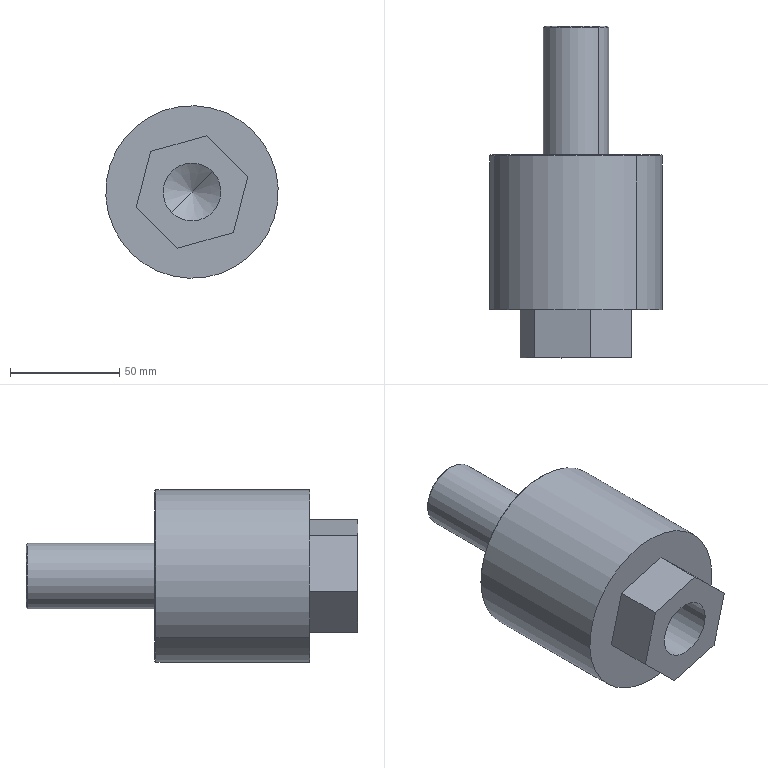Component | SolidWorks | FloatingJointJA140-30-150-1 | 1 solid | 22 faces | box 79 x 152 x 79 mm | volume 405367 mm3 | plane 10 | cylinder 6 | cone 6 | commonest cylinder face diameters 26.5 x2 79 x2 30 x2
STEP:
#1=CARTESIAN_POINT('',(-3.638,47.083,27.291));
#2=VERTEX_POINT('',#1);
#3=CARTESIAN_POINT('',(-4.368,47.083,26.546));
#4=VERTEX_POINT('',#3);
#5=CARTESIAN_POINT('',(-4.003,47.083,26.918));
#6=DIRECTION('',(-0.,-1.,0.));
#7=DIRECTION('',(-0.7002,0.,-0.7139));
#8=AXIS2_PLACEMENT_3D('',#5,#6,#7);
#9=CIRCLE('',#8,0.5217);
#10=EDGE_CURVE('',#2,#4,#9,.T.);
#11=ORIENTED_EDGE('',*,*,#10,.F.);
#12=CARTESIAN_POINT('',(-3.638,45.429,27.291));
#13=VERTEX_POINT('',#12);
#14=CARTESIAN_POINT('',(-3.638,45.429,27.291));
#15=DIRECTION('',(-0.,-1.,0.));
#16=VECTOR('',#15,39.37);
#17=LINE('',#14,#16);
#18=EDGE_CURVE('',#2,#13,#17,.T.);
#19=ORIENTED_EDGE('',*,*,#18,.T.);
#20=CARTESIAN_POINT('',(-4.368,45.429,26.546));
#21=VERTEX_POINT('',#20);
#22=CARTESIAN_POINT('',(-4.003,45.429,26.918));
#23=DIRECTION('',(-0.,-1.,0.));
#24=DIRECTION('',(-0.7002,0.,-0.7139));
#25=AXIS2_PLACEMENT_3D('',#22,#23,#24);
#26=CIRCLE('',#25,0.5217);
#27=EDGE_CURVE('',#13,#21,#26,.T.);
#28=ORIENTED_EDGE('',*,*,#27,.T.);
#29=CARTESIAN_POINT('',(-4.368,45.429,26.546));
#30=DIRECTION('',(-0.,-1.,0.));
#31=VECTOR('',#30,39.37);
#32=LINE('',#29,#31);
#33=EDGE_CURVE('',#4,#21,#32,.T.);
#34=ORIENTED_EDGE('',*,*,#33,.F.);
#35=EDGE_LOOP('',(#11,#19,#28,#34));
#36=FACE_OUTER_BOUND('',#35,.T.);
#37=CARTESIAN_POINT('',(-4.003,45.429,26.918));
#38=DIRECTION('',(-0.,-1.,0.));
#39=DIRECTION('',(-0.7002,0.,-0.7139));
#40=AXIS2_PLACEMENT_3D('',#37,#38,#39);
#41=CYLINDRICAL_SURFACE('',#40,0.5217);
#42=ADVANCED_FACE('',(#36),#41,.F.);
#43=CARTESIAN_POINT('',(-4.003,47.396,26.918));
#44=VERTEX_POINT('',#43);
#45=CARTESIAN_POINT('',(-4.368,47.083,26.546));
#46=DIRECTION('',(-0.6002,-0.515,-0.6119));
#47=VECTOR('',#46,39.37);
#48=LINE('',#45,#47);
#49=EDGE_CURVE('',#44,#4,#48,.T.);
#50=ORIENTED_EDGE('',*,*,#49,.F.);
#51=CARTESIAN_POINT('',(-3.638,47.083,27.291));
#52=DIRECTION('',(0.6002,-0.515,0.6119));
#53=VECTOR('',#52,39.37);
#54=LINE('',#51,#53);
#55=EDGE_CURVE('',#44,#2,#54,.T.);
#56=ORIENTED_EDGE('',*,*,#55,.T.);
#57=ORIENTED_EDGE('',*,*,#10,.T.);
#58=EDGE_LOOP('',(#50,#56,#57));
#59=FACE_OUTER_BOUND('',#58,.T.);
#60=CARTESIAN_POINT('',(-4.003,47.083,26.918));
#61=DIRECTION('',(-0.,-1.,0.));
#62=DIRECTION('',(-0.7002,0.,-0.7139));
#63=AXIS2_PLACEMENT_3D('',#60,#61,#62);
#64=CONICAL_SURFACE('',#63,0.5217,1.03);
#65=ADVANCED_FACE('',(#59),#64,.F.);
#66=CARTESIAN_POINT('',(-3.603,51.413,27.326));
#67=VERTEX_POINT('',#66);
#68=CARTESIAN_POINT('',(-4.403,51.413,26.511));
#69=VERTEX_POINT('',#68);
#70=CARTESIAN_POINT('',(-4.003,51.413,26.918));
#71=DIRECTION('',(0.,1.,-0.));
#72=DIRECTION('',(0.7002,0.,0.7139));
#73=AXIS2_PLACEMENT_3D('',#70,#71,#72);
#74=CIRCLE('',#73,0.5709);
#75=EDGE_CURVE('',#67,#69,#74,.T.);
#76=ORIENTED_EDGE('',*,*,#75,.F.);
#77=CARTESIAN_POINT('',(-3.59,51.394,27.34));
#78=VERTEX_POINT('',#77);
#79=CARTESIAN_POINT('',(-3.59,51.394,27.34));
#80=DIRECTION('',(0.4951,-0.7071,0.5048));
#81=VECTOR('',#80,39.37);
#82=LINE('',#79,#81);
#83=EDGE_CURVE('',#67,#78,#82,.T.);
#84=ORIENTED_EDGE('',*,*,#83,.T.);
#85=CARTESIAN_POINT('',(-4.417,51.394,26.497));
#86=VERTEX_POINT('',#85);
#87=CARTESIAN_POINT('',(-4.003,51.394,26.918));
#88=DIRECTION('',(-0.,-1.,0.));
#89=DIRECTION('',(0.7002,0.,0.7139));
#90=AXIS2_PLACEMENT_3D('',#87,#88,#89);
#91=CIRCLE('',#90,0.5906);
#92=EDGE_CURVE('',#86,#78,#91,.T.);
#93=ORIENTED_EDGE('',*,*,#92,.F.);
#94=CARTESIAN_POINT('',(-4.417,51.394,26.497));
#95=DIRECTION('',(-0.4951,-0.7071,-0.5048));
#96=VECTOR('',#95,39.37);
#97=LINE('',#94,#96);
#98=EDGE_CURVE('',#69,#86,#97,.T.);
#99=ORIENTED_EDGE('',*,*,#98,.F.);
#100=EDGE_LOOP('',(#76,#84,#93,#99));
#101=FACE_OUTER_BOUND('',#100,.T.);
#102=CARTESIAN_POINT('',(-4.003,51.394,26.918));
#103=DIRECTION('',(-0.,-1.,0.));
#104=DIRECTION('',(-0.7002,0.,-0.7139));
#105=AXIS2_PLACEMENT_3D('',#102,#103,#104);
#106=CONICAL_SURFACE('',#105,0.5906,0.7854);
#107=ADVANCED_FACE('',(#101),#106,.T.);
#108=CARTESIAN_POINT('',(-2.928,49.09,28.014));
#109=VERTEX_POINT('',#108);
#110=CARTESIAN_POINT('',(-5.078,49.09,25.822));
#111=VERTEX_POINT('',#110);
#112=CARTESIAN_POINT('',(-4.003,49.09,26.918));
#113=DIRECTION('',(0.,1.,-0.));
#114=DIRECTION('',(0.7002,0.,0.7139));
#115=AXIS2_PLACEMENT_3D('',#112,#113,#114);
#116=CIRCLE('',#115,1.535);
#117=EDGE_CURVE('',#109,#111,#116,.T.);
#118=ORIENTED_EDGE('',*,*,#117,.F.);
#119=CARTESIAN_POINT('',(-2.914,49.071,28.028));
#120=VERTEX_POINT('',#119);
#121=CARTESIAN_POINT('',(-2.914,49.071,28.028));
#122=DIRECTION('',(0.4951,-0.7071,0.5048));
#123=VECTOR('',#122,39.37);
#124=LINE('',#121,#123);
#125=EDGE_CURVE('',#109,#120,#124,.T.);
#126=ORIENTED_EDGE('',*,*,#125,.T.);
#127=CARTESIAN_POINT('',(-5.092,49.071,25.808));
#128=VERTEX_POINT('',#127);
#129=CARTESIAN_POINT('',(-4.003,49.071,26.918));
#130=DIRECTION('',(-0.,-1.,0.));
#131=DIRECTION('',(0.7002,0.,0.7139));
#132=AXIS2_PLACEMENT_3D('',#129,#130,#131);
#133=CIRCLE('',#132,1.555);
#134=EDGE_CURVE('',#128,#120,#133,.T.);
#135=ORIENTED_EDGE('',*,*,#134,.F.);
#136=CARTESIAN_POINT('',(-5.092,49.071,25.808));
#137=DIRECTION('',(-0.4951,-0.7071,-0.5048));
#138=VECTOR('',#137,39.37);
#139=LINE('',#136,#138);
#140=EDGE_CURVE('',#111,#128,#139,.T.);
#141=ORIENTED_EDGE('',*,*,#140,.F.);
#142=EDGE_LOOP('',(#118,#126,#135,#141));
#143=FACE_OUTER_BOUND('',#142,.T.);
#144=CARTESIAN_POINT('',(-4.003,49.071,26.918));
#145=DIRECTION('',(-0.,-1.,0.));
#146=DIRECTION('',(-0.7002,0.,-0.7139));
#147=AXIS2_PLACEMENT_3D('',#144,#145,#146);
#148=CONICAL_SURFACE('',#147,1.555,0.7854);
#149=ADVANCED_FACE('',(#143),#148,.T.);
#150=ORIENTED_EDGE('',*,*,#134,.T.);
#151=CARTESIAN_POINT('',(-2.914,46.295,28.028));
#152=VERTEX_POINT('',#151);
#153=CARTESIAN_POINT('',(-2.914,45.429,28.028));
#154=DIRECTION('',(-0.,-1.,0.));
#155=VECTOR('',#154,39.37);
#156=LINE('',#153,#155);
#157=EDGE_CURVE('',#120,#152,#156,.T.);
#158=ORIENTED_EDGE('',*,*,#157,.T.);
#159=CARTESIAN_POINT('',(-5.092,46.295,25.808));
#160=VERTEX_POINT('',#159);
#161=CARTESIAN_POINT('',(-4.003,46.295,26.918));
#162=DIRECTION('',(-0.,-1.,0.));
#163=DIRECTION('',(-0.7002,0.,-0.7139));
#164=AXIS2_PLACEMENT_3D('',#161,#162,#163);
#165=CIRCLE('',#164,1.555);
#166=EDGE_CURVE('',#160,#152,#165,.T.);
#167=ORIENTED_EDGE('',*,*,#166,.F.);
#168=CARTESIAN_POINT('',(-5.092,45.429,25.808));
#169=DIRECTION('',(-0.,-1.,0.));
#170=VECTOR('',#169,39.37);
#171=LINE('',#168,#170);
#172=EDGE_CURVE('',#128,#160,#171,.T.);
#173=ORIENTED_EDGE('',*,*,#172,.F.);
#174=EDGE_LOOP('',(#150,#158,#167,#173));
#175=FACE_OUTER_BOUND('',#174,.T.);
#176=CARTESIAN_POINT('',(-4.003,45.429,26.918));
#177=DIRECTION('',(-0.,-1.,0.));
#178=DIRECTION('',(-0.7002,0.,-0.7139));
#179=AXIS2_PLACEMENT_3D('',#176,#177,#178);
#180=CYLINDRICAL_SURFACE('',#179,1.555);
#181=ADVANCED_FACE('',(#175),#180,.T.);
#182=ORIENTED_EDGE('',*,*,#92,.T.);
#183=CARTESIAN_POINT('',(-3.59,49.09,27.34));
#184=VERTEX_POINT('',#183);
#185=CARTESIAN_POINT('',(-3.59,45.429,27.34));
#186=DIRECTION('',(-0.,-1.,0.));
#187=VECTOR('',#186,39.37);
#188=LINE('',#185,#187);
#189=EDGE_CURVE('',#78,#184,#188,.T.);
#190=ORIENTED_EDGE('',*,*,#189,.T.);
#191=CARTESIAN_POINT('',(-4.417,49.09,26.497));
#192=VERTEX_POINT('',#191);
#193=CARTESIAN_POINT('',(-4.003,49.09,26.918));
#194=DIRECTION('',(-0.,-1.,0.));
#195=DIRECTION('',(-0.7002,0.,-0.7139));
#196=AXIS2_PLACEMENT_3D('',#193,#194,#195);
#197=CIRCLE('',#196,0.5906);
#198=EDGE_CURVE('',#192,#184,#197,.T.);
#199=ORIENTED_EDGE('',*,*,#198,.F.);
#200=CARTESIAN_POINT('',(-4.417,45.429,26.497));
#201=DIRECTION('',(-0.,-1.,0.));
#202=VECTOR('',#201,39.37);
#203=LINE('',#200,#202);
#204=EDGE_CURVE('',#86,#192,#203,.T.);
#205=ORIENTED_EDGE('',*,*,#204,.F.);
#206=EDGE_LOOP('',(#182,#190,#199,#205));
#207=FACE_OUTER_BOUND('',#206,.T.);
#208=CARTESIAN_POINT('',(-4.003,45.429,26.918));
#209=DIRECTION('',(-0.,-1.,0.));
#210=DIRECTION('',(-0.7002,0.,-0.7139));
#211=AXIS2_PLACEMENT_3D('',#208,#209,#210);
#212=CYLINDRICAL_SURFACE('',#211,0.5906);
#213=ADVANCED_FACE('',(#207),#212,.T.);
#214=CARTESIAN_POINT('',(-4.003,51.413,26.918));
#215=DIRECTION('',(0.,1.,-0.));
#216=DIRECTION('',(0.7002,0.,0.7139));
#217=AXIS2_PLACEMENT_3D('',#214,#215,#216);
#218=CIRCLE('',#217,0.5709);
#219=EDGE_CURVE('',#69,#67,#218,.T.);
#220=ORIENTED_EDGE('',*,*,#219,.T.);
#221=ORIENTED_EDGE('',*,*,#75,.T.);
#222=EDGE_LOOP('',(#220,#221));
#223=FACE_OUTER_BOUND('',#222,.T.);
#224=CARTESIAN_POINT('',(-4.003,51.413,26.918));
#225=DIRECTION('',(0.,1.,-0.));
#226=DIRECTION('',(0.7002,-0.,0.7139));
#227=AXIS2_PLACEMENT_3D('',#224,#225,#226);
#228=PLANE('',#227);
#229=ADVANCED_FACE('',(#223),#228,.T.);
#230=ORIENTED_EDGE('',*,*,#189,.F.);
#231=CARTESIAN_POINT('',(-4.003,51.394,26.918));
#232=DIRECTION('',(-0.,-1.,0.));
#233=DIRECTION('',(0.7002,0.,0.7139));
#234=AXIS2_PLACEMENT_3D('',#231,#232,#233);
#235=CIRCLE('',#234,0.5906);
#236=EDGE_CURVE('',#78,#86,#235,.T.);
#237=ORIENTED_EDGE('',*,*,#236,.T.);
#238=ORIENTED_EDGE('',*,*,#204,.T.);
#239=CARTESIAN_POINT('',(-4.003,49.09,26.918));
#240=DIRECTION('',(-0.,-1.,0.));
#241=DIRECTION('',(-0.7002,0.,-0.7139));
#242=AXIS2_PLACEMENT_3D('',#239,#240,#241);
#243=CIRCLE('',#242,0.5906);
#244=EDGE_CURVE('',#184,#192,#243,.T.);
#245=ORIENTED_EDGE('',*,*,#244,.F.);
#246=EDGE_LOOP('',(#230,#237,#238,#245));
#247=FACE_OUTER_BOUND('',#246,.T.);
#248=CARTESIAN_POINT('',(-4.003,45.429,26.918));
#249=DIRECTION('',(-0.,-1.,0.));
#250=DIRECTION('',(-0.7002,0.,-0.7139));
#251=AXIS2_PLACEMENT_3D('',#248,#249,#250);
#252=CYLINDRICAL_SURFACE('',#251,0.5906);
#253=ADVANCED_FACE('',(#247),#252,.T.);
#254=CARTESIAN_POINT('',(-4.003,49.09,26.918));
#255=DIRECTION('',(0.,1.,-0.));
#256=DIRECTION('',(0.7002,0.,0.7139));
#257=AXIS2_PLACEMENT_3D('',#254,#255,#256);
#258=CIRCLE('',#257,1.535);
#259=EDGE_CURVE('',#111,#109,#258,.T.);
#260=ORIENTED_EDGE('',*,*,#259,.T.);
#261=ORIENTED_EDGE('',*,*,#117,.T.);
#262=EDGE_LOOP('',(#260,#261));
#263=FACE_OUTER_BOUND('',#262,.T.);
#264=ORIENTED_EDGE('',*,*,#198,.T.);
#265=ORIENTED_EDGE('',*,*,#244,.T.);
#266=EDGE_LOOP('',(#264,#265));
#267=FACE_BOUND('',#266,.T.);
#268=CARTESIAN_POINT('',(-5.092,49.09,25.808));
#269=DIRECTION('',(0.,1.,-0.));
#270=DIRECTION('',(0.7002,-0.,0.7139));
#271=AXIS2_PLACEMENT_3D('',#268,#269,#270);
#272=PLANE('',#271);
#273=ADVANCED_FACE('',(#263,#267),#272,.T.);
#274=ORIENTED_EDGE('',*,*,#157,.F.);
#275=CARTESIAN_POINT('',(-4.003,49.071,26.918));
#276=DIRECTION('',(-0.,-1.,0.));
#277=DIRECTION('',(0.7002,0.,0.7139));
#278=AXIS2_PLACEMENT_3D('',#275,#276,#277);
#279=CIRCLE('',#278,1.555);
#280=EDGE_CURVE('',#120,#128,#279,.T.);
#281=ORIENTED_EDGE('',*,*,#280,.T.);
#282=ORIENTED_EDGE('',*,*,#172,.T.);
#283=CARTESIAN_POINT('',(-4.003,46.295,26.918));
#284=DIRECTION('',(-0.,-1.,0.));
#285=DIRECTION('',(-0.7002,0.,-0.7139));
#286=AXIS2_PLACEMENT_3D('',#283,#284,#285);
#287=CIRCLE('',#286,1.555);
#288=EDGE_CURVE('',#152,#160,#287,.T.);
#289=ORIENTED_EDGE('',*,*,#288,.F.);
#290=EDGE_LOOP('',(#274,#281,#282,#289));
#291=FACE_OUTER_BOUND('',#290,.T.);
#292=CARTESIAN_POINT('',(-4.003,45.429,26.918));
#293=DIRECTION('',(-0.,-1.,0.));
#294=DIRECTION('',(-0.7002,0.,-0.7139));
#295=AXIS2_PLACEMENT_3D('',#292,#293,#294);
#296=CYLINDRICAL_SURFACE('',#295,1.555);
#297=ADVANCED_FACE('',(#291),#296,.T.);
#298=ORIENTED_EDGE('',*,*,#166,.T.);
#299=ORIENTED_EDGE('',*,*,#288,.T.);
#300=EDGE_LOOP('',(#298,#299));
#301=FACE_OUTER_BOUND('',#300,.T.);
#302=CARTESIAN_POINT('',(-4.264,46.295,25.906));
#303=VERTEX_POINT('',#302);
#304=CARTESIAN_POINT('',(-3.257,46.295,26.186));
#305=VERTEX_POINT('',#304);
#306=CARTESIAN_POINT('',(-4.264,46.295,25.906));
#307=DIRECTION('',(0.9634,0.,0.2682));
#308=VECTOR('',#307,39.37);
#309=LINE('',#306,#308);
#310=EDGE_CURVE('',#303,#305,#309,.T.);
#311=ORIENTED_EDGE('',*,*,#310,.F.);
#312=CARTESIAN_POINT('',(-5.01,46.295,26.638));
#313=VERTEX_POINT('',#312);
#314=CARTESIAN_POINT('',(-5.01,46.295,26.638));
#315=DIRECTION('',(0.7139,0.,-0.7002));
#316=VECTOR('',#315,39.37);
#317=LINE('',#314,#316);
#318=EDGE_CURVE('',#313,#303,#317,.T.);
#319=ORIENTED_EDGE('',*,*,#318,.F.);
#320=CARTESIAN_POINT('',(-4.75,46.295,27.65));
#321=VERTEX_POINT('',#320);
#322=CARTESIAN_POINT('',(-4.75,46.295,27.65));
#323=DIRECTION('',(-0.2495,0.,-0.9684));
#324=VECTOR('',#323,39.37);
#325=LINE('',#322,#324);
#326=EDGE_CURVE('',#321,#313,#325,.T.);
#327=ORIENTED_EDGE('',*,*,#326,.F.);
#328=CARTESIAN_POINT('',(-3.742,46.295,27.931));
#329=VERTEX_POINT('',#328);
#330=CARTESIAN_POINT('',(-3.742,46.295,27.931));
#331=DIRECTION('',(-0.9634,-0.,-0.2682));
#332=VECTOR('',#331,39.37);
#333=LINE('',#330,#332);
#334=EDGE_CURVE('',#329,#321,#333,.T.);
#335=ORIENTED_EDGE('',*,*,#334,.F.);
#336=CARTESIAN_POINT('',(-2.996,46.295,27.199));
#337=VERTEX_POINT('',#336);
#338=CARTESIAN_POINT('',(-2.996,46.295,27.199));
#339=DIRECTION('',(-0.7139,-0.,0.7002));
#340=VECTOR('',#339,39.37);
#341=LINE('',#338,#340);
#342=EDGE_CURVE('',#337,#329,#341,.T.);
#343=ORIENTED_EDGE('',*,*,#342,.F.);
#344=CARTESIAN_POINT('',(-3.257,46.295,26.186));
#345=DIRECTION('',(0.2495,-0.,0.9684));
#346=VECTOR('',#345,39.37);
#347=LINE('',#344,#346);
#348=EDGE_CURVE('',#305,#337,#347,.T.);
#349=ORIENTED_EDGE('',*,*,#348,.F.);
#350=EDGE_LOOP('',(#311,#319,#327,#335,#343,#349));
#351=FACE_BOUND('',#350,.T.);
#352=CARTESIAN_POINT('',(-5.092,46.295,25.808));
#353=DIRECTION('',(-0.,-1.,0.));
#354=DIRECTION('',(-0.7002,0.,-0.7139));
#355=AXIS2_PLACEMENT_3D('',#352,#353,#354);
#356=PLANE('',#355);
#357=ADVANCED_FACE('',(#301,#351),#356,.T.);
#358=CARTESIAN_POINT('',(-3.257,45.429,26.186));
#359=VERTEX_POINT('',#358);
#360=CARTESIAN_POINT('',(-4.264,45.429,25.906));
#361=VERTEX_POINT('',#360);
#362=CARTESIAN_POINT('',(-4.91,45.429,25.726));
#363=DIRECTION('',(-0.9634,-0.,-0.2682));
#364=VECTOR('',#363,39.37);
#365=LINE('',#362,#364);
#366=EDGE_CURVE('',#359,#361,#365,.T.);
#367=ORIENTED_EDGE('',*,*,#366,.T.);
#368=CARTESIAN_POINT('',(-4.264,44.72,25.906));
#369=DIRECTION('',(0.,1.,-0.));
#370=VECTOR('',#369,39.37);
#371=LINE('',#368,#370);
#372=EDGE_CURVE('',#361,#303,#371,.T.);
#373=ORIENTED_EDGE('',*,*,#372,.T.);
#374=ORIENTED_EDGE('',*,*,#310,.T.);
#375=CARTESIAN_POINT('',(-3.257,44.72,26.186));
#376=DIRECTION('',(0.,1.,-0.));
#377=VECTOR('',#376,39.37);
#378=LINE('',#375,#377);
#379=EDGE_CURVE('',#359,#305,#378,.T.);
#380=ORIENTED_EDGE('',*,*,#379,.F.);
#381=EDGE_LOOP('',(#367,#373,#374,#380));
#382=FACE_OUTER_BOUND('',#381,.T.);
#383=CARTESIAN_POINT('',(-4.264,44.72,25.906));
#384=DIRECTION('',(-0.2682,-0.,0.9634));
#385=DIRECTION('',(-0.9634,-0.,-0.2682));
#386=AXIS2_PLACEMENT_3D('',#383,#384,#385);
#387=PLANE('',#386);
#388=ADVANCED_FACE('',(#382),#387,.F.);
#389=CARTESIAN_POINT('',(-2.996,45.429,27.199));
#390=VERTEX_POINT('',#389);
#391=CARTESIAN_POINT('',(-3.424,45.429,25.537));
#392=DIRECTION('',(-0.2495,0.,-0.9684));
#393=VECTOR('',#392,39.37);
#394=LINE('',#391,#393);
#395=EDGE_CURVE('',#390,#359,#394,.T.);
#396=ORIENTED_EDGE('',*,*,#395,.T.);
#397=ORIENTED_EDGE('',*,*,#379,.T.);
#398=ORIENTED_EDGE('',*,*,#348,.T.);
#399=CARTESIAN_POINT('',(-2.996,44.72,27.199));
#400=DIRECTION('',(0.,1.,-0.));
#401=VECTOR('',#400,39.37);
#402=LINE('',#399,#401);
#403=EDGE_CURVE('',#390,#337,#402,.T.);
#404=ORIENTED_EDGE('',*,*,#403,.F.);
#405=EDGE_LOOP('',(#396,#397,#398,#404));
#406=FACE_OUTER_BOUND('',#405,.T.);
#407=CARTESIAN_POINT('',(-3.257,44.72,26.186));
#408=DIRECTION('',(-0.9684,-0.,0.2495));
#409=DIRECTION('',(-0.2495,0.,-0.9684));
#410=AXIS2_PLACEMENT_3D('',#407,#408,#409);
#411=PLANE('',#410);
#412=ADVANCED_FACE('',(#406),#411,.F.);
#413=CARTESIAN_POINT('',(-3.742,45.429,27.931));
#414=VERTEX_POINT('',#413);
#415=CARTESIAN_POINT('',(-3.369,45.429,27.565));
#416=DIRECTION('',(0.7139,0.,-0.7002));
#417=VECTOR('',#416,39.37);
#418=LINE('',#415,#417);
#419=EDGE_CURVE('',#414,#390,#418,.T.);
#420=ORIENTED_EDGE('',*,*,#419,.T.);
#421=ORIENTED_EDGE('',*,*,#403,.T.);
#422=ORIENTED_EDGE('',*,*,#342,.T.);
#423=CARTESIAN_POINT('',(-3.742,44.72,27.931));
#424=DIRECTION('',(0.,1.,-0.));
#425=VECTOR('',#424,39.37);
#426=LINE('',#423,#425);
#427=EDGE_CURVE('',#414,#329,#426,.T.);
#428=ORIENTED_EDGE('',*,*,#427,.F.);
#429=EDGE_LOOP('',(#420,#421,#422,#428));
#430=FACE_OUTER_BOUND('',#429,.T.);
#431=CARTESIAN_POINT('',(-2.996,44.72,27.199));
#432=DIRECTION('',(-0.7002,-0.,-0.7139));
#433=DIRECTION('',(0.,1.,-0.));
#434=AXIS2_PLACEMENT_3D('',#431,#432,#433);
#435=PLANE('',#434);
#436=ADVANCED_FACE('',(#430),#435,.F.);
#437=CARTESIAN_POINT('',(-4.75,45.429,27.65));
#438=VERTEX_POINT('',#437);
#439=CARTESIAN_POINT('',(-5.396,45.429,27.471));
#440=DIRECTION('',(0.9634,0.,0.2682));
#441=VECTOR('',#440,39.37);
#442=LINE('',#439,#441);
#443=EDGE_CURVE('',#438,#414,#442,.T.);
#444=ORIENTED_EDGE('',*,*,#443,.T.);
#445=ORIENTED_EDGE('',*,*,#427,.T.);
#446=ORIENTED_EDGE('',*,*,#334,.T.);
#447=CARTESIAN_POINT('',(-4.75,44.72,27.65));
#448=DIRECTION('',(0.,1.,-0.));
#449=VECTOR('',#448,39.37);
#450=LINE('',#447,#449);
#451=EDGE_CURVE('',#438,#321,#450,.T.);
#452=ORIENTED_EDGE('',*,*,#451,.F.);
#453=EDGE_LOOP('',(#444,#445,#446,#452));
#454=FACE_OUTER_BOUND('',#453,.T.);
#455=CARTESIAN_POINT('',(-3.742,44.72,27.931));
#456=DIRECTION('',(0.2682,0.,-0.9634));
#457=DIRECTION('',(0.9634,0.,0.2682));
#458=AXIS2_PLACEMENT_3D('',#455,#456,#457);
#459=PLANE('',#458);
#460=ADVANCED_FACE('',(#454),#459,.F.);
#461=CARTESIAN_POINT('',(-5.01,45.429,26.638));
#462=VERTEX_POINT('',#461);
#463=CARTESIAN_POINT('',(-5.178,45.429,25.988));
#464=DIRECTION('',(0.2495,-0.,0.9684));
#465=VECTOR('',#464,39.37);
#466=LINE('',#463,#465);
#467=EDGE_CURVE('',#462,#438,#466,.T.);
#468=ORIENTED_EDGE('',*,*,#467,.T.);
#469=ORIENTED_EDGE('',*,*,#451,.T.);
#470=ORIENTED_EDGE('',*,*,#326,.T.);
#471=CARTESIAN_POINT('',(-5.01,44.72,26.638));
#472=DIRECTION('',(0.,1.,-0.));
#473=VECTOR('',#472,39.37);
#474=LINE('',#471,#473);
#475=EDGE_CURVE('',#462,#313,#474,.T.);
#476=ORIENTED_EDGE('',*,*,#475,.F.);
#477=EDGE_LOOP('',(#468,#469,#470,#476));
#478=FACE_OUTER_BOUND('',#477,.T.);
#479=CARTESIAN_POINT('',(-4.75,44.72,27.65));
#480=DIRECTION('',(0.9684,0.,-0.2495));
#481=DIRECTION('',(0.2495,-0.,0.9684));
#482=AXIS2_PLACEMENT_3D('',#479,#480,#481);
#483=PLANE('',#482);
#484=ADVANCED_FACE('',(#478),#483,.F.);
#485=CARTESIAN_POINT('',(-4.637,45.429,26.272));
#486=DIRECTION('',(-0.7139,-0.,0.7002));
#487=VECTOR('',#486,39.37);
#488=LINE('',#485,#487);
#489=EDGE_CURVE('',#361,#462,#488,.T.);
#490=ORIENTED_EDGE('',*,*,#489,.T.);
#491=ORIENTED_EDGE('',*,*,#475,.T.);
#492=ORIENTED_EDGE('',*,*,#318,.T.);
#493=ORIENTED_EDGE('',*,*,#372,.F.);
#494=EDGE_LOOP('',(#490,#491,#492,#493));
#495=FACE_OUTER_BOUND('',#494,.T.);
#496=CARTESIAN_POINT('',(-5.01,44.72,26.638));
#497=DIRECTION('',(0.7002,0.,0.7139));
#498=DIRECTION('',(-0.,-1.,0.));
#499=AXIS2_PLACEMENT_3D('',#496,#497,#498);
#500=PLANE('',#499);
#501=ADVANCED_FACE('',(#495),#500,.F.);
#502=CARTESIAN_POINT('',(-4.003,45.429,26.918));
#503=DIRECTION('',(-0.,-1.,0.));
#504=DIRECTION('',(-0.7002,0.,-0.7139));
#505=AXIS2_PLACEMENT_3D('',#502,#503,#504);
#506=CIRCLE('',#505,0.5217);
#507=EDGE_CURVE('',#21,#13,#506,.T.);
#508=ORIENTED_EDGE('',*,*,#507,.F.);
#509=ORIENTED_EDGE('',*,*,#27,.F.);
#510=EDGE_LOOP('',(#508,#509));
#511=FACE_BOUND('',#510,.T.);
#512=ORIENTED_EDGE('',*,*,#366,.F.);
#513=ORIENTED_EDGE('',*,*,#395,.F.);
#514=ORIENTED_EDGE('',*,*,#419,.F.);
#515=ORIENTED_EDGE('',*,*,#443,.F.);
#516=ORIENTED_EDGE('',*,*,#467,.F.);
#517=ORIENTED_EDGE('',*,*,#489,.F.);
#518=EDGE_LOOP('',(#512,#513,#514,#515,#516,#517));
#519=FACE_OUTER_BOUND('',#518,.T.);
#520=CARTESIAN_POINT('',(-4.968,45.429,25.934));
#521=DIRECTION('',(-0.,-1.,0.));
#522=DIRECTION('',(-0.7002,0.,-0.7139));
#523=AXIS2_PLACEMENT_3D('',#520,#521,#522);
#524=PLANE('',#523);
#525=ADVANCED_FACE('',(#511,#519),#524,.T.);
#526=ORIENTED_EDGE('',*,*,#125,.F.);
#527=ORIENTED_EDGE('',*,*,#259,.F.);
#528=ORIENTED_EDGE('',*,*,#140,.T.);
#529=ORIENTED_EDGE('',*,*,#280,.F.);
#530=EDGE_LOOP('',(#526,#527,#528,#529));
#531=FACE_OUTER_BOUND('',#530,.T.);
#532=CARTESIAN_POINT('',(-4.003,49.071,26.918));
#533=DIRECTION('',(-0.,-1.,0.));
#534=DIRECTION('',(-0.7002,0.,-0.7139));
#535=AXIS2_PLACEMENT_3D('',#532,#533,#534);
#536=CONICAL_SURFACE('',#535,1.555,0.7854);
#537=ADVANCED_FACE('',(#531),#536,.T.);
#538=ORIENTED_EDGE('',*,*,#83,.F.);
#539=ORIENTED_EDGE('',*,*,#219,.F.);
#540=ORIENTED_EDGE('',*,*,#98,.T.);
#541=ORIENTED_EDGE('',*,*,#236,.F.);
#542=EDGE_LOOP('',(#538,#539,#540,#541));
#543=FACE_OUTER_BOUND('',#542,.T.);
#544=CARTESIAN_POINT('',(-4.003,51.394,26.918));
#545=DIRECTION('',(-0.,-1.,0.));
#546=DIRECTION('',(-0.7002,0.,-0.7139));
#547=AXIS2_PLACEMENT_3D('',#544,#545,#546);
#548=CONICAL_SURFACE('',#547,0.5906,0.7854);
#549=ADVANCED_FACE('',(#543),#548,.T.);
#550=ORIENTED_EDGE('',*,*,#55,.F.);
#551=ORIENTED_EDGE('',*,*,#49,.T.);
#552=CARTESIAN_POINT('',(-4.003,47.083,26.918));
#553=DIRECTION('',(-0.,-1.,0.));
#554=DIRECTION('',(-0.7002,0.,-0.7139));
#555=AXIS2_PLACEMENT_3D('',#552,#553,#554);
#556=CIRCLE('',#555,0.5217);
#557=EDGE_CURVE('',#4,#2,#556,.T.);
#558=ORIENTED_EDGE('',*,*,#557,.T.);
#559=EDGE_LOOP('',(#550,#551,#558));
#560=FACE_OUTER_BOUND('',#559,.T.);
#561=CARTESIAN_POINT('',(-4.003,47.083,26.918));
#562=DIRECTION('',(-0.,-1.,0.));
#563=DIRECTION('',(-0.7002,0.,-0.7139));
#564=AXIS2_PLACEMENT_3D('',#561,#562,#563);
#565=CONICAL_SURFACE('',#564,0.5217,1.03);
#566=ADVANCED_FACE('',(#560),#565,.F.);
#567=ORIENTED_EDGE('',*,*,#18,.F.);
#568=ORIENTED_EDGE('',*,*,#557,.F.);
#569=ORIENTED_EDGE('',*,*,#33,.T.);
#570=ORIENTED_EDGE('',*,*,#507,.T.);
#571=EDGE_LOOP('',(#567,#568,#569,#570));
#572=FACE_OUTER_BOUND('',#571,.T.);
#573=CARTESIAN_POINT('',(-4.003,45.429,26.918));
#574=DIRECTION('',(-0.,-1.,0.));
#575=DIRECTION('',(-0.7002,0.,-0.7139));
#576=AXIS2_PLACEMENT_3D('',#573,#574,#575);
#577=CYLINDRICAL_SURFACE('',#576,0.5217);
#578=ADVANCED_FACE('',(#572),#577,.F.);
#579=CLOSED_SHELL('',(#42,#65,#107,#149,#181,#213,#229,#253,#273,#297,#357,#388,#412,#436,#460,#484,#501,#525,#537,#549,#566,#578));
#580=MANIFOLD_SOLID_BREP('',#579);
#581=CARTESIAN_POINT('',(0.,0.,0.));
#582=DIRECTION('',(0.,0.,1.));
#583=DIRECTION('',(1.,0.,0.));
#584=AXIS2_PLACEMENT_3D('',#581,#582,#583);
#585=(LENGTH_UNIT()NAMED_UNIT(*)SI_UNIT($,.METRE.));
#586=LENGTH_MEASURE_WITH_UNIT(LENGTH_MEASURE(0.0254),#585);
#587=DIMENSIONAL_EXPONENTS(1.,0.,0.,0.,0.,0.,0.);
#588=(CONVERSION_BASED_UNIT('',#586)LENGTH_UNIT()NAMED_UNIT(#587));
#589=UNCERTAINTY_MEASURE_WITH_UNIT(LENGTH_MEASURE(0.00001),#588,'','');
#590=(NAMED_UNIT(*)PLANE_ANGLE_UNIT()SI_UNIT($,.RADIAN.));
#591=(NAMED_UNIT(*)SI_UNIT($,.STERADIAN.)SOLID_ANGLE_UNIT());
#592=(GEOMETRIC_REPRESENTATION_CONTEXT(3)GLOBAL_UNCERTAINTY_ASSIGNED_CONTEXT((#589))GLOBAL_UNIT_ASSIGNED_CONTEXT((#588,#590,#591))REPRESENTATION_CONTEXT('',''));
#593=ADVANCED_BREP_SHAPE_REPRESENTATION('',(#580,#584),#592);
#594=COLOUR_RGB('',0.7922,0.8196,0.9333);
#595=FILL_AREA_STYLE_COLOUR('',#594);
#596=FILL_AREA_STYLE('',(#595));
#597=SURFACE_STYLE_FILL_AREA(#596);
#598=SURFACE_SIDE_STYLE('',(#597));
#599=SURFACE_STYLE_USAGE(.BOTH.,#598);
#600=PRESENTATION_STYLE_ASSIGNMENT((#599));
#601=STYLED_ITEM('',(#600),#580);
#602=PRESENTATION_LAYER_ASSIGNMENT('','',(#601));
#603=(LENGTH_UNIT()NAMED_UNIT(*)SI_UNIT($,.METRE.));
#604=LENGTH_MEASURE_WITH_UNIT(LENGTH_MEASURE(0.0254),#603);
#605=DIMENSIONAL_EXPONENTS(1.,0.,0.,0.,0.,0.,0.);
#606=(CONVERSION_BASED_UNIT('',#604)LENGTH_UNIT()NAMED_UNIT(#605));
#607=UNCERTAINTY_MEASURE_WITH_UNIT(LENGTH_MEASURE(0.00001),#606,'','');
#608=(NAMED_UNIT(*)PLANE_ANGLE_UNIT()SI_UNIT($,.RADIAN.));
#609=(NAMED_UNIT(*)SI_UNIT($,.STERADIAN.)SOLID_ANGLE_UNIT());
#610=(GEOMETRIC_REPRESENTATION_CONTEXT(3)GLOBAL_UNCERTAINTY_ASSIGNED_CONTEXT((#607))GLOBAL_UNIT_ASSIGNED_CONTEXT((#606,#608,#609))REPRESENTATION_CONTEXT('',''));
#611=MECHANICAL_DESIGN_GEOMETRIC_PRESENTATION_REPRESENTATION('',(#601),#610);